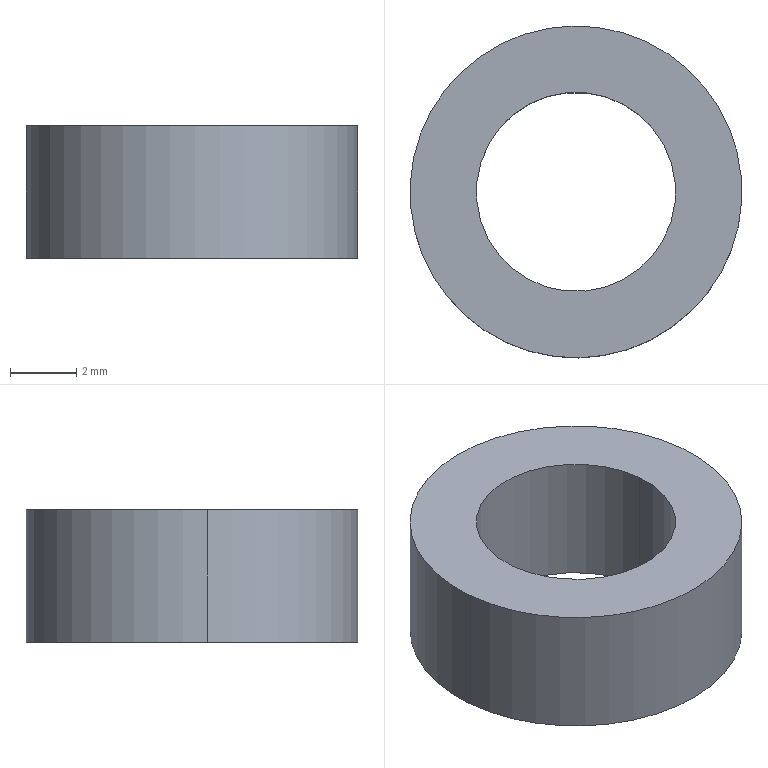Component | SolidWorks | 9-1 | 1 solid | 6 faces | box 10 x 10 x 4 mm | volume 201 mm3 | cylinder 4 | plane 2 | commonest cylinder face diameters 6 x2 10 x2
build123d program:
from build123d import *

# Parameters (mm, degrees)
SKETCH1_R           = 5
SKETCH1_R_2         = 3
BOSS_EXTRUDE1_DEPTH = 4


with BuildPart() as part:
    # Sketch1 → Boss-Extrude1 (new body)
    with BuildSketch(Plane.XY):
        Circle(SKETCH1_R)
        Circle(SKETCH1_R_2, mode=Mode.SUBTRACT)
    extrude(amount=BOSS_EXTRUDE1_DEPTH)


solid = part.part

# Placed as in the assembly
solid = solid.moved(Location((69.329, 7.034, -22.938), (0, 0, 0)))
STEP:
#1=COLOUR_RGB('',0.7922,0.8196,0.9333);
#2=FILL_AREA_STYLE_COLOUR('',#1);
#3=FILL_AREA_STYLE('',(#2));
#4=SURFACE_STYLE_FILL_AREA(#3);
#5=SURFACE_SIDE_STYLE('',(#4));
#6=SURFACE_STYLE_USAGE(.BOTH.,#5);
#7=PRESENTATION_STYLE_ASSIGNMENT((#6));
#8=CARTESIAN_POINT('',(2.612,0.266,-0.7456));
#9=VERTEX_POINT('',#8);
#10=CARTESIAN_POINT('',(2.847,0.2879,-0.7456));
#11=VERTEX_POINT('',#10);
#12=CARTESIAN_POINT('',(2.73,0.2769,-0.7456));
#13=DIRECTION('',(0.,0.,1.));
#14=DIRECTION('',(0.9957,0.09249,0.));
#15=AXIS2_PLACEMENT_3D('',#12,#13,#14);
#16=CIRCLE('',#15,0.1181);
#17=EDGE_CURVE('',#9,#11,#16,.T.);
#18=ORIENTED_EDGE('',*,*,#17,.T.);
#19=CARTESIAN_POINT('',(2.847,0.2879,-0.9031));
#20=VERTEX_POINT('',#19);
#21=CARTESIAN_POINT('',(2.847,0.2879,-0.7456));
#22=DIRECTION('',(0.,0.,-1.));
#23=VECTOR('',#22,39.37);
#24=LINE('',#21,#23);
#25=EDGE_CURVE('',#11,#20,#24,.T.);
#26=ORIENTED_EDGE('',*,*,#25,.T.);
#27=CARTESIAN_POINT('',(2.612,0.266,-0.9031));
#28=VERTEX_POINT('',#27);
#29=CARTESIAN_POINT('',(2.73,0.2769,-0.9031));
#30=DIRECTION('',(0.,0.,1.));
#31=DIRECTION('',(0.9957,0.09249,0.));
#32=AXIS2_PLACEMENT_3D('',#29,#30,#31);
#33=CIRCLE('',#32,0.1181);
#34=EDGE_CURVE('',#28,#20,#33,.T.);
#35=ORIENTED_EDGE('',*,*,#34,.F.);
#36=CARTESIAN_POINT('',(2.612,0.266,-0.7456));
#37=DIRECTION('',(0.,0.,-1.));
#38=VECTOR('',#37,39.37);
#39=LINE('',#36,#38);
#40=EDGE_CURVE('',#9,#28,#39,.T.);
#41=ORIENTED_EDGE('',*,*,#40,.F.);
#42=EDGE_LOOP('',(#18,#26,#35,#41));
#43=FACE_OUTER_BOUND('',#42,.T.);
#44=CARTESIAN_POINT('',(2.73,0.2769,-0.7456));
#45=DIRECTION('',(0.,0.,-1.));
#46=DIRECTION('',(-0.9957,-0.09249,0.));
#47=AXIS2_PLACEMENT_3D('',#44,#45,#46);
#48=CYLINDRICAL_SURFACE('',#47,0.1181);
#49=ADVANCED_FACE('',(#43),#48,.F.);
#50=CARTESIAN_POINT('',(2.926,0.2951,-0.7456));
#51=VERTEX_POINT('',#50);
#52=CARTESIAN_POINT('',(2.533,0.2587,-0.7456));
#53=VERTEX_POINT('',#52);
#54=CARTESIAN_POINT('',(2.73,0.2769,-0.7456));
#55=DIRECTION('',(0.,0.,1.));
#56=DIRECTION('',(0.9957,0.09249,0.));
#57=AXIS2_PLACEMENT_3D('',#54,#55,#56);
#58=CIRCLE('',#57,0.1969);
#59=EDGE_CURVE('',#51,#53,#58,.T.);
#60=ORIENTED_EDGE('',*,*,#59,.F.);
#61=CARTESIAN_POINT('',(2.926,0.2951,-0.9031));
#62=VERTEX_POINT('',#61);
#63=CARTESIAN_POINT('',(2.926,0.2951,-0.7456));
#64=DIRECTION('',(0.,0.,-1.));
#65=VECTOR('',#64,39.37);
#66=LINE('',#63,#65);
#67=EDGE_CURVE('',#51,#62,#66,.T.);
#68=ORIENTED_EDGE('',*,*,#67,.T.);
#69=CARTESIAN_POINT('',(2.533,0.2587,-0.9031));
#70=VERTEX_POINT('',#69);
#71=CARTESIAN_POINT('',(2.73,0.2769,-0.9031));
#72=DIRECTION('',(0.,0.,1.));
#73=DIRECTION('',(0.9957,0.09249,0.));
#74=AXIS2_PLACEMENT_3D('',#71,#72,#73);
#75=CIRCLE('',#74,0.1969);
#76=EDGE_CURVE('',#62,#70,#75,.T.);
#77=ORIENTED_EDGE('',*,*,#76,.T.);
#78=CARTESIAN_POINT('',(2.533,0.2587,-0.7456));
#79=DIRECTION('',(0.,0.,-1.));
#80=VECTOR('',#79,39.37);
#81=LINE('',#78,#80);
#82=EDGE_CURVE('',#53,#70,#81,.T.);
#83=ORIENTED_EDGE('',*,*,#82,.F.);
#84=EDGE_LOOP('',(#60,#68,#77,#83));
#85=FACE_OUTER_BOUND('',#84,.T.);
#86=CARTESIAN_POINT('',(2.73,0.2769,-0.7456));
#87=DIRECTION('',(0.,0.,-1.));
#88=DIRECTION('',(-0.9957,-0.09249,0.));
#89=AXIS2_PLACEMENT_3D('',#86,#87,#88);
#90=CYLINDRICAL_SURFACE('',#89,0.1969);
#91=ADVANCED_FACE('',(#85),#90,.T.);
#92=CARTESIAN_POINT('',(2.73,0.2769,-0.7456));
#93=DIRECTION('',(0.,0.,1.));
#94=DIRECTION('',(0.9957,0.09249,0.));
#95=AXIS2_PLACEMENT_3D('',#92,#93,#94);
#96=CIRCLE('',#95,0.1969);
#97=EDGE_CURVE('',#53,#51,#96,.T.);
#98=ORIENTED_EDGE('',*,*,#97,.T.);
#99=ORIENTED_EDGE('',*,*,#59,.T.);
#100=EDGE_LOOP('',(#98,#99));
#101=FACE_OUTER_BOUND('',#100,.T.);
#102=ORIENTED_EDGE('',*,*,#17,.F.);
#103=CARTESIAN_POINT('',(2.73,0.2769,-0.7456));
#104=DIRECTION('',(0.,0.,1.));
#105=DIRECTION('',(0.9957,0.09249,0.));
#106=AXIS2_PLACEMENT_3D('',#103,#104,#105);
#107=CIRCLE('',#106,0.1181);
#108=EDGE_CURVE('',#11,#9,#107,.T.);
#109=ORIENTED_EDGE('',*,*,#108,.F.);
#110=EDGE_LOOP('',(#102,#109));
#111=FACE_BOUND('',#110,.T.);
#112=CARTESIAN_POINT('',(2.73,0.2769,-0.7456));
#113=DIRECTION('',(0.,0.,1.));
#114=DIRECTION('',(0.9957,0.09249,0.));
#115=AXIS2_PLACEMENT_3D('',#112,#113,#114);
#116=PLANE('',#115);
#117=ADVANCED_FACE('',(#101,#111),#116,.T.);
#118=CARTESIAN_POINT('',(2.73,0.2769,-0.9031));
#119=DIRECTION('',(0.,0.,1.));
#120=DIRECTION('',(0.9957,0.09249,0.));
#121=AXIS2_PLACEMENT_3D('',#118,#119,#120);
#122=CIRCLE('',#121,0.1969);
#123=EDGE_CURVE('',#70,#62,#122,.T.);
#124=ORIENTED_EDGE('',*,*,#123,.F.);
#125=ORIENTED_EDGE('',*,*,#76,.F.);
#126=EDGE_LOOP('',(#124,#125));
#127=FACE_OUTER_BOUND('',#126,.T.);
#128=ORIENTED_EDGE('',*,*,#34,.T.);
#129=CARTESIAN_POINT('',(2.73,0.2769,-0.9031));
#130=DIRECTION('',(0.,0.,1.));
#131=DIRECTION('',(0.9957,0.09249,0.));
#132=AXIS2_PLACEMENT_3D('',#129,#130,#131);
#133=CIRCLE('',#132,0.1181);
#134=EDGE_CURVE('',#20,#28,#133,.T.);
#135=ORIENTED_EDGE('',*,*,#134,.T.);
#136=EDGE_LOOP('',(#128,#135));
#137=FACE_BOUND('',#136,.T.);
#138=CARTESIAN_POINT('',(2.73,0.2769,-0.9031));
#139=DIRECTION('',(0.,0.,1.));
#140=DIRECTION('',(0.9957,0.09249,0.));
#141=AXIS2_PLACEMENT_3D('',#138,#139,#140);
#142=PLANE('',#141);
#143=ADVANCED_FACE('',(#127,#137),#142,.F.);
#144=ORIENTED_EDGE('',*,*,#67,.F.);
#145=ORIENTED_EDGE('',*,*,#97,.F.);
#146=ORIENTED_EDGE('',*,*,#82,.T.);
#147=ORIENTED_EDGE('',*,*,#123,.T.);
#148=EDGE_LOOP('',(#144,#145,#146,#147));
#149=FACE_OUTER_BOUND('',#148,.T.);
#150=CARTESIAN_POINT('',(2.73,0.2769,-0.7456));
#151=DIRECTION('',(0.,0.,-1.));
#152=DIRECTION('',(-0.9957,-0.09249,0.));
#153=AXIS2_PLACEMENT_3D('',#150,#151,#152);
#154=CYLINDRICAL_SURFACE('',#153,0.1969);
#155=ADVANCED_FACE('',(#149),#154,.T.);
#156=ORIENTED_EDGE('',*,*,#25,.F.);
#157=ORIENTED_EDGE('',*,*,#108,.T.);
#158=ORIENTED_EDGE('',*,*,#40,.T.);
#159=ORIENTED_EDGE('',*,*,#134,.F.);
#160=EDGE_LOOP('',(#156,#157,#158,#159));
#161=FACE_OUTER_BOUND('',#160,.T.);
#162=CARTESIAN_POINT('',(2.73,0.2769,-0.7456));
#163=DIRECTION('',(0.,0.,-1.));
#164=DIRECTION('',(-0.9957,-0.09249,0.));
#165=AXIS2_PLACEMENT_3D('',#162,#163,#164);
#166=CYLINDRICAL_SURFACE('',#165,0.1181);
#167=ADVANCED_FACE('',(#161),#166,.F.);
#168=CLOSED_SHELL('',(#49,#91,#117,#143,#155,#167));
#169=MANIFOLD_SOLID_BREP('',#168);
#170=STYLED_ITEM('',(#7),#169);
#171=PRESENTATION_LAYER_ASSIGNMENT('','',(#170));
#172=(LENGTH_UNIT()NAMED_UNIT(*)SI_UNIT($,.METRE.));
#173=LENGTH_MEASURE_WITH_UNIT(LENGTH_MEASURE(0.0254),#172);
#174=DIMENSIONAL_EXPONENTS(1.,0.,0.,0.,0.,0.,0.);
#175=(CONVERSION_BASED_UNIT('',#173)LENGTH_UNIT()NAMED_UNIT(#174));
#176=UNCERTAINTY_MEASURE_WITH_UNIT(LENGTH_MEASURE(0.00001),#175,'','');
#177=(NAMED_UNIT(*)PLANE_ANGLE_UNIT()SI_UNIT($,.RADIAN.));
#178=(NAMED_UNIT(*)SI_UNIT($,.STERADIAN.)SOLID_ANGLE_UNIT());
#179=(GEOMETRIC_REPRESENTATION_CONTEXT(3)GLOBAL_UNCERTAINTY_ASSIGNED_CONTEXT((#176))GLOBAL_UNIT_ASSIGNED_CONTEXT((#175,#177,#178))REPRESENTATION_CONTEXT('',''));
#180=MECHANICAL_DESIGN_GEOMETRIC_PRESENTATION_REPRESENTATION('',(#170),#179);
#181=CARTESIAN_POINT('',(0.,0.,0.));
#182=DIRECTION('',(0.,0.,1.));
#183=DIRECTION('',(1.,0.,0.));
#184=AXIS2_PLACEMENT_3D('',#181,#182,#183);
#185=(LENGTH_UNIT()NAMED_UNIT(*)SI_UNIT($,.METRE.));
#186=LENGTH_MEASURE_WITH_UNIT(LENGTH_MEASURE(0.0254),#185);
#187=DIMENSIONAL_EXPONENTS(1.,0.,0.,0.,0.,0.,0.);
#188=(CONVERSION_BASED_UNIT('',#186)LENGTH_UNIT()NAMED_UNIT(#187));
#189=UNCERTAINTY_MEASURE_WITH_UNIT(LENGTH_MEASURE(0.00001),#188,'','');
#190=(NAMED_UNIT(*)PLANE_ANGLE_UNIT()SI_UNIT($,.RADIAN.));
#191=(NAMED_UNIT(*)SI_UNIT($,.STERADIAN.)SOLID_ANGLE_UNIT());
#192=(GEOMETRIC_REPRESENTATION_CONTEXT(3)GLOBAL_UNCERTAINTY_ASSIGNED_CONTEXT((#189))GLOBAL_UNIT_ASSIGNED_CONTEXT((#188,#190,#191))REPRESENTATION_CONTEXT('',''));
#193=ADVANCED_BREP_SHAPE_REPRESENTATION('',(#169,#184),#192);